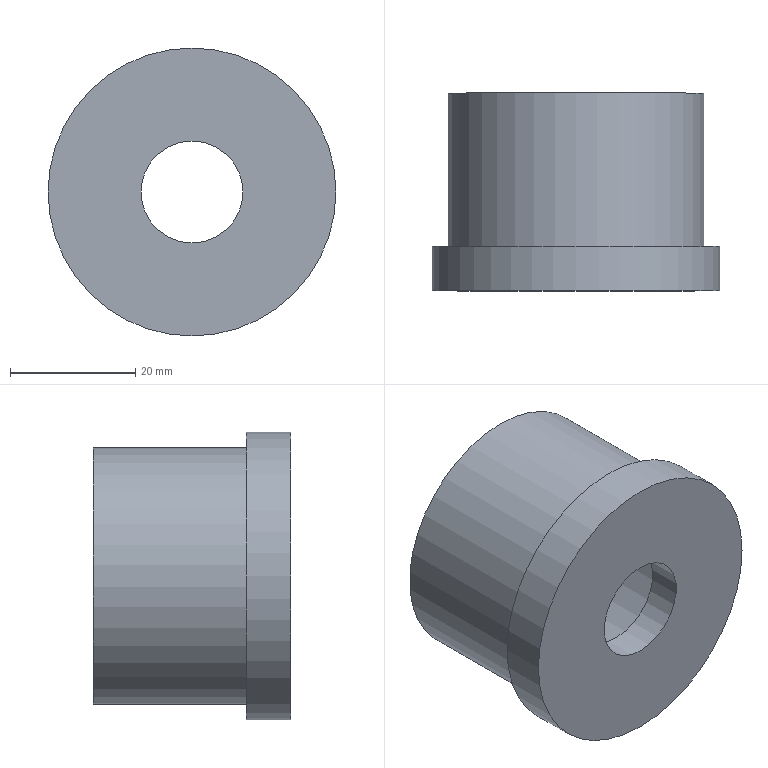Component | NX | BUSHING | 1 solid | 8 faces | box 46 x 31.6 x 46 mm | volume 17747 mm3 | plane 4 | cylinder 4 | commonest cylinder face diameters 16.298 x1 35 x1 41 x1 46 x1
STEP:
#1=CARTESIAN_POINT('',(0.,0.,0.));
#2=DIRECTION('',(0.,0.,1.));
#3=DIRECTION('',(1.,0.,0.));
#4=AXIS2_PLACEMENT_3D('',#1,#2,#3);
#5=CARTESIAN_POINT('',(0.,31.4,-8.149));
#6=VERTEX_POINT('',#5);
#7=CARTESIAN_POINT('',(0.,31.4,0.));
#8=DIRECTION('',(0.,-1.,0.));
#9=DIRECTION('',(0.,0.,-1.));
#10=AXIS2_PLACEMENT_3D('',#7,#8,#9);
#11=CIRCLE('',#10,8.149);
#12=CARTESIAN_POINT('',(0.,31.4,23.));
#13=DIRECTION('',(0.,1.,0.));
#14=DIRECTION('',(0.,0.,1.));
#15=AXIS2_PLACEMENT_3D('',#12,#13,#14);
#16=PLANE('',#15);
#17=CARTESIAN_POINT('',(-31.149,0.));
#18=CARTESIAN_POINT('',(-31.149,14.114));
#19=CARTESIAN_POINT('',(-18.926,7.057));
#20=CARTESIAN_POINT('',(-6.702,0.));
#21=CARTESIAN_POINT('',(-18.926,-7.057));
#22=CARTESIAN_POINT('',(-31.149,-14.114));
#23=CARTESIAN_POINT('',(-31.149,0.));
#24=(BOUNDED_CURVE()B_SPLINE_CURVE(2,(#17,#18,#19,#20,#21,#22,#23),.UNSPECIFIED.,.T.,.F.)B_SPLINE_CURVE_WITH_KNOTS((1,2,2,2,2,1),(-2.094,0.,2.094,4.189,6.283,8.378),.UNSPECIFIED.)CURVE()GEOMETRIC_REPRESENTATION_ITEM()RATIONAL_B_SPLINE_CURVE((1.,0.5,1.,0.5,1.,0.5,1.))REPRESENTATION_ITEM(''));
#25=(GEOMETRIC_REPRESENTATION_CONTEXT(2)PARAMETRIC_REPRESENTATION_CONTEXT()REPRESENTATION_CONTEXT('',''));
#26=DEFINITIONAL_REPRESENTATION('',(#24),#25);
#27=PCURVE('',#16,#26);
#28=CARTESIAN_POINT('',(0.,85.313,0.));
#29=DIRECTION('',(0.,-1.,0.));
#30=DIRECTION('',(0.,0.,-1.));
#31=AXIS2_PLACEMENT_3D('',#28,#29,#30);
#32=CYLINDRICAL_SURFACE('',#31,8.149);
#33=CARTESIAN_POINT('',(0.,53.913));
#34=DIRECTION('',(1.,0.));
#35=VECTOR('',#34,1.);
#36=LINE('',#33,#35);
#37=(GEOMETRIC_REPRESENTATION_CONTEXT(2)PARAMETRIC_REPRESENTATION_CONTEXT()REPRESENTATION_CONTEXT('',''));
#38=DEFINITIONAL_REPRESENTATION('',(#36),#37);
#39=PCURVE('',#32,#38);
#40=SURFACE_CURVE('',#11,(#27,#39),.PCURVE_S1.);
#41=EDGE_CURVE('',#6,#6,#40,.T.);
#42=ORIENTED_EDGE('',*,*,#41,.F.);
#43=EDGE_LOOP('',(#42));
#44=FACE_BOUND('',#43,.T.);
#45=CARTESIAN_POINT('',(0.,31.4,-23.));
#46=VERTEX_POINT('',#45);
#47=CARTESIAN_POINT('',(0.,31.4,0.));
#48=DIRECTION('',(0.,-1.,0.));
#49=DIRECTION('',(0.,0.,-1.));
#50=AXIS2_PLACEMENT_3D('',#47,#48,#49);
#51=CIRCLE('',#50,23.);
#52=CARTESIAN_POINT('',(-46.,0.));
#53=CARTESIAN_POINT('',(-46.,39.837));
#54=CARTESIAN_POINT('',(-11.5,19.919));
#55=CARTESIAN_POINT('',(23.,0.));
#56=CARTESIAN_POINT('',(-11.5,-19.919));
#57=CARTESIAN_POINT('',(-46.,-39.837));
#58=CARTESIAN_POINT('',(-46.,0.));
#59=(BOUNDED_CURVE()B_SPLINE_CURVE(2,(#52,#53,#54,#55,#56,#57,#58),.UNSPECIFIED.,.T.,.F.)B_SPLINE_CURVE_WITH_KNOTS((1,2,2,2,2,1),(-2.094,0.,2.094,4.189,6.283,8.378),.UNSPECIFIED.)CURVE()GEOMETRIC_REPRESENTATION_ITEM()RATIONAL_B_SPLINE_CURVE((1.,0.5,1.,0.5,1.,0.5,1.))REPRESENTATION_ITEM(''));
#60=(GEOMETRIC_REPRESENTATION_CONTEXT(2)PARAMETRIC_REPRESENTATION_CONTEXT()REPRESENTATION_CONTEXT('',''));
#61=DEFINITIONAL_REPRESENTATION('',(#59),#60);
#62=PCURVE('',#16,#61);
#63=CARTESIAN_POINT('',(0.,85.313,0.));
#64=DIRECTION('',(0.,-1.,0.));
#65=DIRECTION('',(0.,0.,-1.));
#66=AXIS2_PLACEMENT_3D('',#63,#64,#65);
#67=CYLINDRICAL_SURFACE('',#66,23.);
#68=CARTESIAN_POINT('',(0.,53.913));
#69=DIRECTION('',(1.,0.));
#70=VECTOR('',#69,1.);
#71=LINE('',#68,#70);
#72=(GEOMETRIC_REPRESENTATION_CONTEXT(2)PARAMETRIC_REPRESENTATION_CONTEXT()REPRESENTATION_CONTEXT('',''));
#73=DEFINITIONAL_REPRESENTATION('',(#71),#72);
#74=PCURVE('',#67,#73);
#75=SURFACE_CURVE('',#51,(#62,#74),.PCURVE_S1.);
#76=EDGE_CURVE('',#46,#46,#75,.T.);
#77=ORIENTED_EDGE('',*,*,#76,.T.);
#78=EDGE_LOOP('',(#77));
#79=FACE_BOUND('',#78,.T.);
#80=ADVANCED_FACE('',(#44,#79),#16,.F.);
#81=CARTESIAN_POINT('',(0.,36.714,-8.149));
#82=VERTEX_POINT('',#81);
#83=CARTESIAN_POINT('',(0.,36.714,0.));
#84=DIRECTION('',(0.,-1.,0.));
#85=DIRECTION('',(0.,0.,-1.));
#86=AXIS2_PLACEMENT_3D('',#83,#84,#85);
#87=CIRCLE('',#86,8.149);
#88=CARTESIAN_POINT('',(0.,48.599));
#89=DIRECTION('',(1.,0.));
#90=VECTOR('',#89,1.);
#91=LINE('',#88,#90);
#92=(GEOMETRIC_REPRESENTATION_CONTEXT(2)PARAMETRIC_REPRESENTATION_CONTEXT()REPRESENTATION_CONTEXT('',''));
#93=DEFINITIONAL_REPRESENTATION('',(#91),#92);
#94=PCURVE('',#32,#93);
#95=CARTESIAN_POINT('',(0.,36.714,8.149));
#96=DIRECTION('',(0.,-1.,0.));
#97=DIRECTION('',(0.,0.,-1.));
#98=AXIS2_PLACEMENT_3D('',#95,#96,#97);
#99=PLANE('',#98);
#100=CARTESIAN_POINT('',(8.149,0.));
#101=DIRECTION('',(1.,0.));
#102=AXIS2_PLACEMENT_2D('',#100,#101);
#103=CIRCLE('',#102,8.149);
#104=(GEOMETRIC_REPRESENTATION_CONTEXT(2)PARAMETRIC_REPRESENTATION_CONTEXT()REPRESENTATION_CONTEXT('',''));
#105=DEFINITIONAL_REPRESENTATION('',(#103),#104);
#106=PCURVE('',#99,#105);
#107=SURFACE_CURVE('',#87,(#94,#106),.PCURVE_S1.);
#108=EDGE_CURVE('',#82,#82,#107,.T.);
#109=ORIENTED_EDGE('',*,*,#108,.T.);
#110=CARTESIAN_POINT('',(0.,36.714,-8.149));
#111=CARTESIAN_POINT('',(0.,31.4,-8.149));
#112=B_SPLINE_CURVE_WITH_KNOTS('',1,(#110,#111),.UNSPECIFIED.,.F.,.F.,(2,2),(48.599,53.913),.PIECEWISE_BEZIER_KNOTS.);
#113=CARTESIAN_POINT('',(6.283,0.));
#114=DIRECTION('',(0.,1.));
#115=VECTOR('',#114,1.);
#116=LINE('',#113,#115);
#117=(GEOMETRIC_REPRESENTATION_CONTEXT(2)PARAMETRIC_REPRESENTATION_CONTEXT()REPRESENTATION_CONTEXT('',''));
#118=DEFINITIONAL_REPRESENTATION('',(#116),#117);
#119=PCURVE('',#32,#118);
#120=CARTESIAN_POINT('',(0.,0.));
#121=DIRECTION('',(0.,1.));
#122=VECTOR('',#121,1.);
#123=LINE('',#120,#122);
#124=(GEOMETRIC_REPRESENTATION_CONTEXT(2)PARAMETRIC_REPRESENTATION_CONTEXT()REPRESENTATION_CONTEXT('',''));
#125=DEFINITIONAL_REPRESENTATION('',(#123),#124);
#126=PCURVE('',#32,#125);
#127=SEAM_CURVE('',#112,(#119,#126),.PCURVE_S1.);
#128=EDGE_CURVE('',#82,#6,#127,.T.);
#129=ORIENTED_EDGE('',*,*,#128,.T.);
#130=ORIENTED_EDGE('',*,*,#41,.F.);
#131=ORIENTED_EDGE('',*,*,#128,.F.);
#132=EDGE_LOOP('',(#109,#129,#130,#131));
#133=FACE_BOUND('',#132,.F.);
#134=ADVANCED_FACE('',(#133),#32,.F.);
#135=CARTESIAN_POINT('',(0.,36.714,-17.5));
#136=VERTEX_POINT('',#135);
#137=CARTESIAN_POINT('',(0.,36.714,0.));
#138=DIRECTION('',(0.,-1.,0.));
#139=DIRECTION('',(0.,0.,-1.));
#140=AXIS2_PLACEMENT_3D('',#137,#138,#139);
#141=CIRCLE('',#140,17.5);
#142=CARTESIAN_POINT('',(8.149,0.));
#143=DIRECTION('',(1.,0.));
#144=AXIS2_PLACEMENT_2D('',#142,#143);
#145=CIRCLE('',#144,17.5);
#146=(GEOMETRIC_REPRESENTATION_CONTEXT(2)PARAMETRIC_REPRESENTATION_CONTEXT()REPRESENTATION_CONTEXT('',''));
#147=DEFINITIONAL_REPRESENTATION('',(#145),#146);
#148=PCURVE('',#99,#147);
#149=CARTESIAN_POINT('',(0.,85.313,0.));
#150=DIRECTION('',(0.,-1.,0.));
#151=DIRECTION('',(0.,0.,-1.));
#152=AXIS2_PLACEMENT_3D('',#149,#150,#151);
#153=CYLINDRICAL_SURFACE('',#152,17.5);
#154=CARTESIAN_POINT('',(0.,48.599));
#155=DIRECTION('',(1.,0.));
#156=VECTOR('',#155,1.);
#157=LINE('',#154,#156);
#158=(GEOMETRIC_REPRESENTATION_CONTEXT(2)PARAMETRIC_REPRESENTATION_CONTEXT()REPRESENTATION_CONTEXT('',''));
#159=DEFINITIONAL_REPRESENTATION('',(#157),#158);
#160=PCURVE('',#153,#159);
#161=SURFACE_CURVE('',#141,(#148,#160),.PCURVE_S1.);
#162=EDGE_CURVE('',#136,#136,#161,.T.);
#163=ORIENTED_EDGE('',*,*,#162,.F.);
#164=EDGE_LOOP('',(#163));
#165=FACE_BOUND('',#164,.T.);
#166=ORIENTED_EDGE('',*,*,#108,.T.);
#167=EDGE_LOOP('',(#166));
#168=FACE_BOUND('',#167,.T.);
#169=ADVANCED_FACE('',(#165,#168),#99,.F.);
#170=CARTESIAN_POINT('',(0.,63.,-17.5));
#171=VERTEX_POINT('',#170);
#172=CARTESIAN_POINT('',(0.,63.,0.));
#173=DIRECTION('',(0.,-1.,0.));
#174=DIRECTION('',(0.,0.,-1.));
#175=AXIS2_PLACEMENT_3D('',#172,#173,#174);
#176=CIRCLE('',#175,17.5);
#177=CARTESIAN_POINT('',(0.,22.313));
#178=DIRECTION('',(1.,0.));
#179=VECTOR('',#178,1.);
#180=LINE('',#177,#179);
#181=(GEOMETRIC_REPRESENTATION_CONTEXT(2)PARAMETRIC_REPRESENTATION_CONTEXT()REPRESENTATION_CONTEXT('',''));
#182=DEFINITIONAL_REPRESENTATION('',(#180),#181);
#183=PCURVE('',#153,#182);
#184=CARTESIAN_POINT('',(0.,63.,17.5));
#185=DIRECTION('',(0.,-1.,0.));
#186=DIRECTION('',(0.,0.,-1.));
#187=AXIS2_PLACEMENT_3D('',#184,#185,#186);
#188=PLANE('',#187);
#189=CARTESIAN_POINT('',(17.5,0.));
#190=DIRECTION('',(1.,0.));
#191=AXIS2_PLACEMENT_2D('',#189,#190);
#192=CIRCLE('',#191,17.5);
#193=(GEOMETRIC_REPRESENTATION_CONTEXT(2)PARAMETRIC_REPRESENTATION_CONTEXT()REPRESENTATION_CONTEXT('',''));
#194=DEFINITIONAL_REPRESENTATION('',(#192),#193);
#195=PCURVE('',#188,#194);
#196=SURFACE_CURVE('',#176,(#183,#195),.PCURVE_S1.);
#197=EDGE_CURVE('',#171,#171,#196,.T.);
#198=ORIENTED_EDGE('',*,*,#197,.T.);
#199=CARTESIAN_POINT('',(0.,63.,-17.5));
#200=CARTESIAN_POINT('',(0.,36.714,-17.5));
#201=B_SPLINE_CURVE_WITH_KNOTS('',1,(#199,#200),.UNSPECIFIED.,.F.,.F.,(2,2),(22.313,48.599),.PIECEWISE_BEZIER_KNOTS.);
#202=CARTESIAN_POINT('',(6.283,0.));
#203=DIRECTION('',(0.,1.));
#204=VECTOR('',#203,1.);
#205=LINE('',#202,#204);
#206=(GEOMETRIC_REPRESENTATION_CONTEXT(2)PARAMETRIC_REPRESENTATION_CONTEXT()REPRESENTATION_CONTEXT('',''));
#207=DEFINITIONAL_REPRESENTATION('',(#205),#206);
#208=PCURVE('',#153,#207);
#209=CARTESIAN_POINT('',(0.,0.));
#210=DIRECTION('',(0.,1.));
#211=VECTOR('',#210,1.);
#212=LINE('',#209,#211);
#213=(GEOMETRIC_REPRESENTATION_CONTEXT(2)PARAMETRIC_REPRESENTATION_CONTEXT()REPRESENTATION_CONTEXT('',''));
#214=DEFINITIONAL_REPRESENTATION('',(#212),#213);
#215=PCURVE('',#153,#214);
#216=SEAM_CURVE('',#201,(#208,#215),.PCURVE_S1.);
#217=EDGE_CURVE('',#171,#136,#216,.T.);
#218=ORIENTED_EDGE('',*,*,#217,.T.);
#219=ORIENTED_EDGE('',*,*,#162,.F.);
#220=ORIENTED_EDGE('',*,*,#217,.F.);
#221=EDGE_LOOP('',(#198,#218,#219,#220));
#222=FACE_BOUND('',#221,.F.);
#223=ADVANCED_FACE('',(#222),#153,.F.);
#224=CARTESIAN_POINT('',(0.,63.,-20.5));
#225=VERTEX_POINT('',#224);
#226=CARTESIAN_POINT('',(0.,63.,0.));
#227=DIRECTION('',(0.,-1.,0.));
#228=DIRECTION('',(0.,0.,-1.));
#229=AXIS2_PLACEMENT_3D('',#226,#227,#228);
#230=CIRCLE('',#229,20.5);
#231=CARTESIAN_POINT('',(17.5,0.));
#232=DIRECTION('',(1.,0.));
#233=AXIS2_PLACEMENT_2D('',#231,#232);
#234=CIRCLE('',#233,20.5);
#235=(GEOMETRIC_REPRESENTATION_CONTEXT(2)PARAMETRIC_REPRESENTATION_CONTEXT()REPRESENTATION_CONTEXT('',''));
#236=DEFINITIONAL_REPRESENTATION('',(#234),#235);
#237=PCURVE('',#188,#236);
#238=CARTESIAN_POINT('',(0.,85.313,0.));
#239=DIRECTION('',(0.,-1.,0.));
#240=DIRECTION('',(0.,0.,-1.));
#241=AXIS2_PLACEMENT_3D('',#238,#239,#240);
#242=CYLINDRICAL_SURFACE('',#241,20.5);
#243=CARTESIAN_POINT('',(0.,22.313));
#244=DIRECTION('',(1.,0.));
#245=VECTOR('',#244,1.);
#246=LINE('',#243,#245);
#247=(GEOMETRIC_REPRESENTATION_CONTEXT(2)PARAMETRIC_REPRESENTATION_CONTEXT()REPRESENTATION_CONTEXT('',''));
#248=DEFINITIONAL_REPRESENTATION('',(#246),#247);
#249=PCURVE('',#242,#248);
#250=SURFACE_CURVE('',#230,(#237,#249),.PCURVE_S1.);
#251=EDGE_CURVE('',#225,#225,#250,.T.);
#252=ORIENTED_EDGE('',*,*,#251,.F.);
#253=EDGE_LOOP('',(#252));
#254=FACE_BOUND('',#253,.T.);
#255=ORIENTED_EDGE('',*,*,#197,.T.);
#256=EDGE_LOOP('',(#255));
#257=FACE_BOUND('',#256,.T.);
#258=ADVANCED_FACE('',(#254,#257),#188,.F.);
#259=CARTESIAN_POINT('',(0.,38.5,-20.5));
#260=VERTEX_POINT('',#259);
#261=CARTESIAN_POINT('',(0.,38.5,0.));
#262=DIRECTION('',(0.,-1.,0.));
#263=DIRECTION('',(0.,0.,-1.));
#264=AXIS2_PLACEMENT_3D('',#261,#262,#263);
#265=CIRCLE('',#264,20.5);
#266=CARTESIAN_POINT('',(0.,46.813));
#267=DIRECTION('',(1.,0.));
#268=VECTOR('',#267,1.);
#269=LINE('',#266,#268);
#270=(GEOMETRIC_REPRESENTATION_CONTEXT(2)PARAMETRIC_REPRESENTATION_CONTEXT()REPRESENTATION_CONTEXT('',''));
#271=DEFINITIONAL_REPRESENTATION('',(#269),#270);
#272=PCURVE('',#242,#271);
#273=CARTESIAN_POINT('',(0.,38.5,20.5));
#274=DIRECTION('',(0.,-1.,0.));
#275=DIRECTION('',(0.,0.,-1.));
#276=AXIS2_PLACEMENT_3D('',#273,#274,#275);
#277=PLANE('',#276);
#278=CARTESIAN_POINT('',(20.5,0.));
#279=DIRECTION('',(1.,0.));
#280=AXIS2_PLACEMENT_2D('',#278,#279);
#281=CIRCLE('',#280,20.5);
#282=(GEOMETRIC_REPRESENTATION_CONTEXT(2)PARAMETRIC_REPRESENTATION_CONTEXT()REPRESENTATION_CONTEXT('',''));
#283=DEFINITIONAL_REPRESENTATION('',(#281),#282);
#284=PCURVE('',#277,#283);
#285=SURFACE_CURVE('',#265,(#272,#284),.PCURVE_S1.);
#286=EDGE_CURVE('',#260,#260,#285,.T.);
#287=ORIENTED_EDGE('',*,*,#286,.F.);
#288=CARTESIAN_POINT('',(-0.,63.,-20.5));
#289=CARTESIAN_POINT('',(-0.,38.5,-20.5));
#290=B_SPLINE_CURVE_WITH_KNOTS('',1,(#288,#289),.UNSPECIFIED.,.F.,.F.,(2,2),(22.313,46.813),.PIECEWISE_BEZIER_KNOTS.);
#291=CARTESIAN_POINT('',(0.,0.));
#292=DIRECTION('',(0.,1.));
#293=VECTOR('',#292,1.);
#294=LINE('',#291,#293);
#295=(GEOMETRIC_REPRESENTATION_CONTEXT(2)PARAMETRIC_REPRESENTATION_CONTEXT()REPRESENTATION_CONTEXT('',''));
#296=DEFINITIONAL_REPRESENTATION('',(#294),#295);
#297=PCURVE('',#242,#296);
#298=CARTESIAN_POINT('',(6.283,0.));
#299=DIRECTION('',(0.,1.));
#300=VECTOR('',#299,1.);
#301=LINE('',#298,#300);
#302=(GEOMETRIC_REPRESENTATION_CONTEXT(2)PARAMETRIC_REPRESENTATION_CONTEXT()REPRESENTATION_CONTEXT('',''));
#303=DEFINITIONAL_REPRESENTATION('',(#301),#302);
#304=PCURVE('',#242,#303);
#305=SEAM_CURVE('',#290,(#297,#304),.PCURVE_S1.);
#306=EDGE_CURVE('',#225,#260,#305,.T.);
#307=ORIENTED_EDGE('',*,*,#306,.F.);
#308=ORIENTED_EDGE('',*,*,#251,.T.);
#309=ORIENTED_EDGE('',*,*,#306,.T.);
#310=EDGE_LOOP('',(#287,#307,#308,#309));
#311=FACE_BOUND('',#310,.T.);
#312=ADVANCED_FACE('',(#311),#242,.T.);
#313=CARTESIAN_POINT('',(0.,38.5,-23.));
#314=VERTEX_POINT('',#313);
#315=CARTESIAN_POINT('',(0.,38.5,0.));
#316=DIRECTION('',(0.,-1.,0.));
#317=DIRECTION('',(0.,0.,-1.));
#318=AXIS2_PLACEMENT_3D('',#315,#316,#317);
#319=CIRCLE('',#318,23.);
#320=CARTESIAN_POINT('',(20.5,0.));
#321=DIRECTION('',(1.,0.));
#322=AXIS2_PLACEMENT_2D('',#320,#321);
#323=CIRCLE('',#322,23.);
#324=(GEOMETRIC_REPRESENTATION_CONTEXT(2)PARAMETRIC_REPRESENTATION_CONTEXT()REPRESENTATION_CONTEXT('',''));
#325=DEFINITIONAL_REPRESENTATION('',(#323),#324);
#326=PCURVE('',#277,#325);
#327=CARTESIAN_POINT('',(0.,46.813));
#328=DIRECTION('',(1.,0.));
#329=VECTOR('',#328,1.);
#330=LINE('',#327,#329);
#331=(GEOMETRIC_REPRESENTATION_CONTEXT(2)PARAMETRIC_REPRESENTATION_CONTEXT()REPRESENTATION_CONTEXT('',''));
#332=DEFINITIONAL_REPRESENTATION('',(#330),#331);
#333=PCURVE('',#67,#332);
#334=SURFACE_CURVE('',#319,(#326,#333),.PCURVE_S1.);
#335=EDGE_CURVE('',#314,#314,#334,.T.);
#336=ORIENTED_EDGE('',*,*,#335,.F.);
#337=EDGE_LOOP('',(#336));
#338=FACE_BOUND('',#337,.T.);
#339=ORIENTED_EDGE('',*,*,#286,.T.);
#340=EDGE_LOOP('',(#339));
#341=FACE_BOUND('',#340,.T.);
#342=ADVANCED_FACE('',(#338,#341),#277,.F.);
#343=ORIENTED_EDGE('',*,*,#76,.F.);
#344=CARTESIAN_POINT('',(-0.,38.5,-23.));
#345=CARTESIAN_POINT('',(-0.,31.4,-23.));
#346=B_SPLINE_CURVE_WITH_KNOTS('',1,(#344,#345),.UNSPECIFIED.,.F.,.F.,(2,2),(46.813,53.913),.PIECEWISE_BEZIER_KNOTS.);
#347=CARTESIAN_POINT('',(0.,0.));
#348=DIRECTION('',(0.,1.));
#349=VECTOR('',#348,1.);
#350=LINE('',#347,#349);
#351=(GEOMETRIC_REPRESENTATION_CONTEXT(2)PARAMETRIC_REPRESENTATION_CONTEXT()REPRESENTATION_CONTEXT('',''));
#352=DEFINITIONAL_REPRESENTATION('',(#350),#351);
#353=PCURVE('',#67,#352);
#354=CARTESIAN_POINT('',(6.283,0.));
#355=DIRECTION('',(0.,1.));
#356=VECTOR('',#355,1.);
#357=LINE('',#354,#356);
#358=(GEOMETRIC_REPRESENTATION_CONTEXT(2)PARAMETRIC_REPRESENTATION_CONTEXT()REPRESENTATION_CONTEXT('',''));
#359=DEFINITIONAL_REPRESENTATION('',(#357),#358);
#360=PCURVE('',#67,#359);
#361=SEAM_CURVE('',#346,(#353,#360),.PCURVE_S1.);
#362=EDGE_CURVE('',#314,#46,#361,.T.);
#363=ORIENTED_EDGE('',*,*,#362,.F.);
#364=ORIENTED_EDGE('',*,*,#335,.T.);
#365=ORIENTED_EDGE('',*,*,#362,.T.);
#366=EDGE_LOOP('',(#343,#363,#364,#365));
#367=FACE_BOUND('',#366,.T.);
#368=ADVANCED_FACE('',(#367),#67,.T.);
#369=CLOSED_SHELL('',(#80,#134,#169,#223,#258,#312,#342,#368));
#370=MANIFOLD_SOLID_BREP('',#369);
#371=(LENGTH_UNIT()NAMED_UNIT(*)SI_UNIT(.MILLI.,.METRE.));
#372=UNCERTAINTY_MEASURE_WITH_UNIT(LENGTH_MEASURE(0.00001),#371,'','');
#373=(NAMED_UNIT(*)PLANE_ANGLE_UNIT()SI_UNIT($,.RADIAN.));
#374=(NAMED_UNIT(*)SI_UNIT($,.STERADIAN.)SOLID_ANGLE_UNIT());
#375=(GEOMETRIC_REPRESENTATION_CONTEXT(3)GLOBAL_UNCERTAINTY_ASSIGNED_CONTEXT((#372))GLOBAL_UNIT_ASSIGNED_CONTEXT((#371,#373,#374))REPRESENTATION_CONTEXT('',''));
#376=ADVANCED_BREP_SHAPE_REPRESENTATION('',(#4,#370),#375);